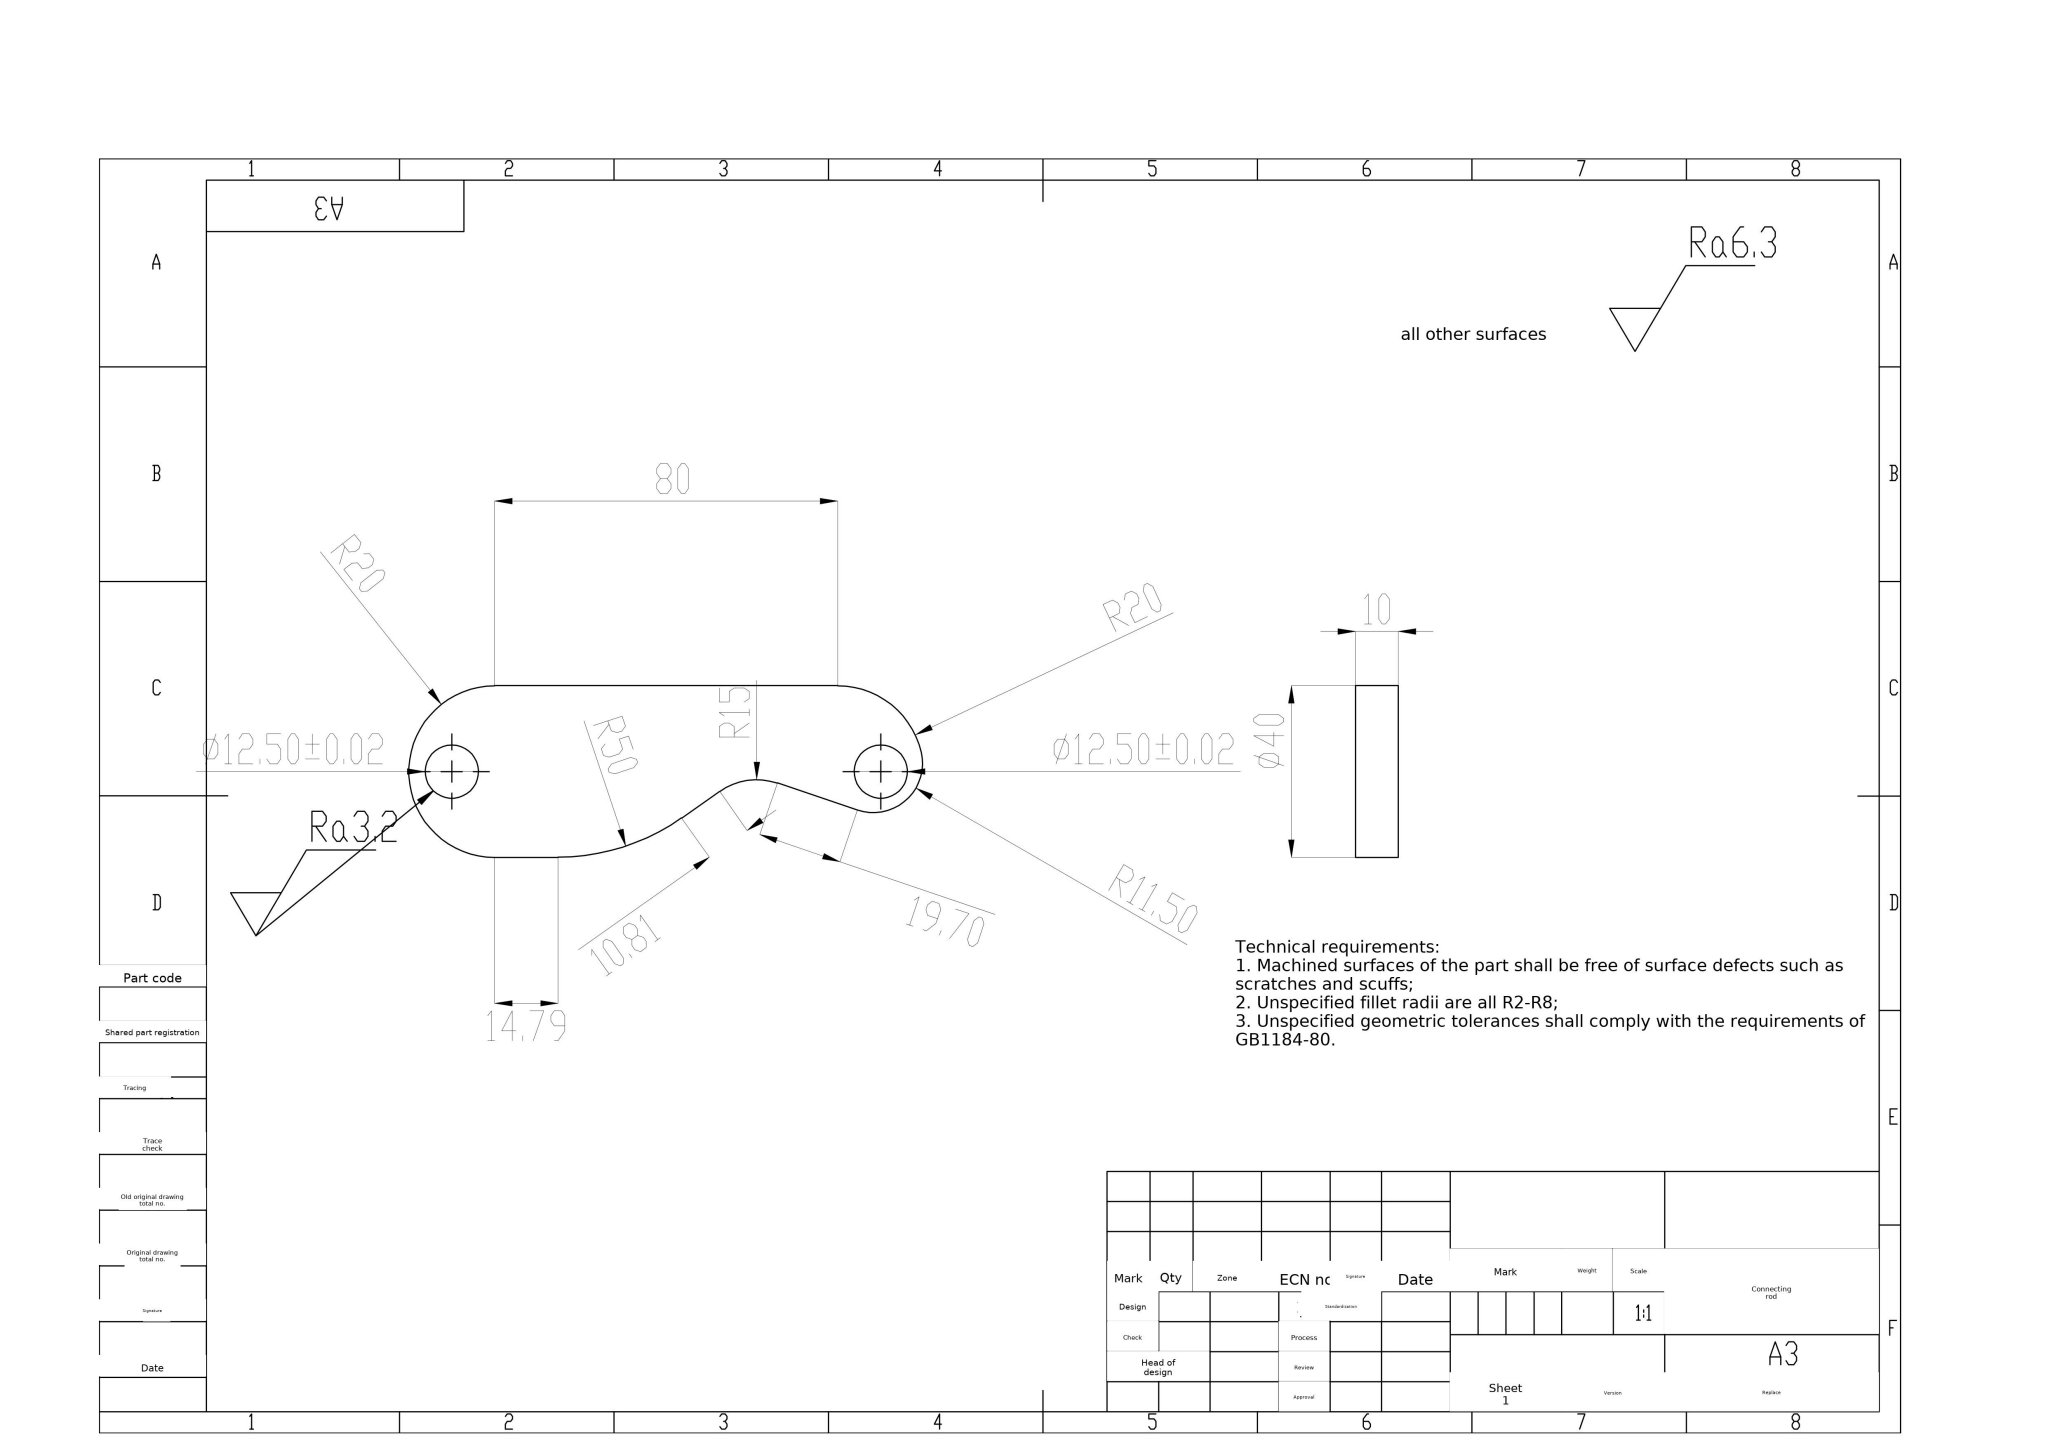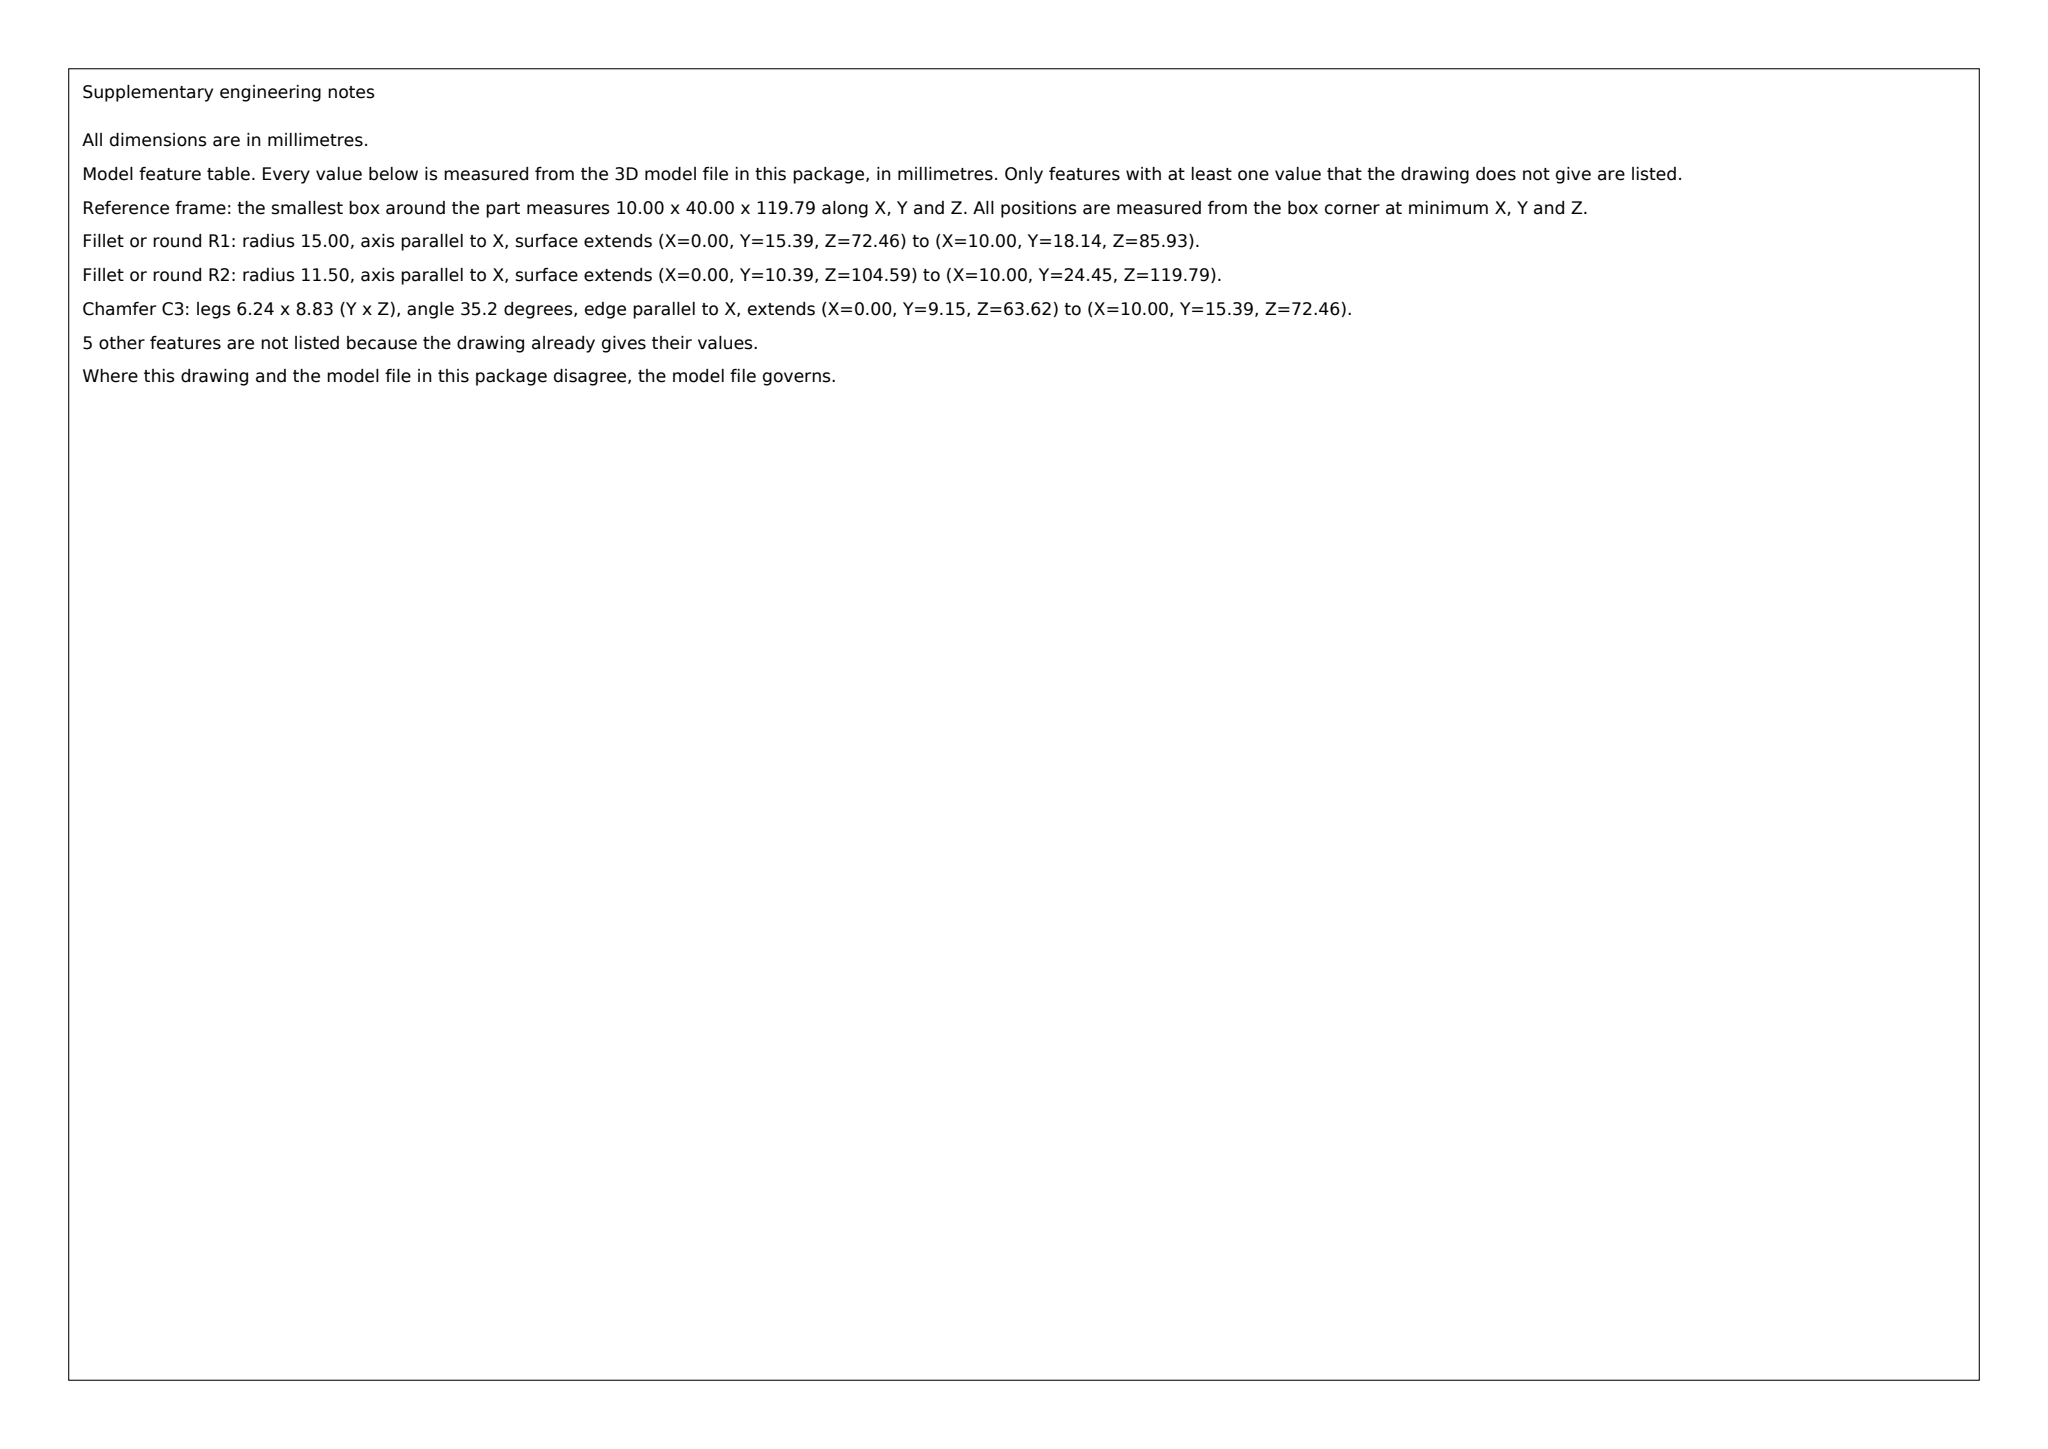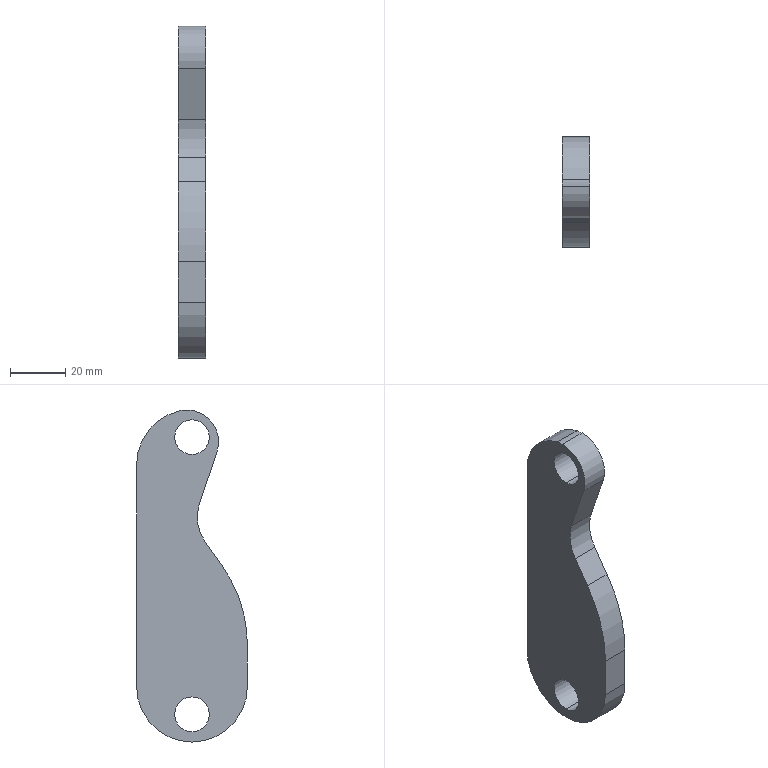Part | SolidWorks | mm | 1 solid | 16 faces | box 10 x 40 x 119.79 mm | volume 34125 mm3 | cylinder 10 | plane 6 | commonest cylinder face diameters 12.5 x4 23 x2 40 x2 30 x1 100 x1
build123d program:
from build123d import *

# Parameters (mm, degrees)
SKETCH1_R           = 1.25
BOSS_EXTRUDE1_DEPTH = 2
CUT_EXTRUDE1_DEPTH  = 13.806
FILLET1_R           = 10
FILLET2_R           = 2.3
SCALE1_SCALE        = 10
SCALE2_SCALE        = 10
SCALE3_SCALE        = 0.1
SCALE4_SCALE        = 0.5


with BuildPart() as part:
    # Sketch1 → Boss-Extrude1 (new body)
    with BuildSketch(Plane(origin=(0, 0, 0), x_dir=(0, 0, -1), z_dir=(1, 0, 0))):
        with BuildLine():
            Line((8, -4), (-8, -4))
            ThreePointArc((-8, -4), (-12, 0), (-8, 4))
            Line((-8, 4), (8, 4))
            ThreePointArc((8, 4), (12, 0), (8, -4))
        make_face()
        with Locations((10, 0)):
            Circle(SKETCH1_R, mode=Mode.SUBTRACT)
        with Locations(Location((-10, 0, 0), (0, 0, 180))):
            Circle(SKETCH1_R, mode=Mode.SUBTRACT)
    extrude(amount=BOSS_EXTRUDE1_DEPTH)

    # Sketch2 → Cut-Extrude1 (cut, through all)
    with BuildSketch(Plane.ZY):
        with BuildLine():
            Line((-1.868, -4), (2.491, -0.9222))
            ThreePointArc((2.491, -0.9222), (3.792, -0.4039), (5.186, -0.5324))
            Line((5.186, -0.5324), (13.896, -3.49))
            Line((13.896, -3.49), (11.205, -5.288))
            Line((11.205, -5.288), (0.9404, -6.462))
            Line((0.9404, -6.462), (-1.868, -4))
        make_face()
    extrude(amount=-CUT_EXTRUDE1_DEPTH, mode=Mode.SUBTRACT)

    # Fillet1
    fillet1_edges = [part.edges().sort_by_distance(p)[0] for p in [
        (1, -4, -1.868),
    ]]
    fillet(fillet1_edges, radius=FILLET1_R)

    # Fillet2
    fillet2_edges = [part.edges().sort_by_distance(p)[0] for p in [
        (1, -2.538, 11.092),
    ]]
    fillet(fillet2_edges, radius=FILLET2_R)


with BuildPart() as part_1:
    # Scale1: scaled about (1, 0.5999, -1.156)
    add(part.part.scale(SCALE1_SCALE).moved(Location((-9, -5.399, 10.403))))


with BuildPart() as part_2:
    # Scale2: scaled about (0, 0, 0)
    add(part_1.part.scale(SCALE2_SCALE))


with BuildPart() as part_3:
    # Scale3: scaled about (0, 0, 0)
    add(part_2.part.scale(SCALE3_SCALE))


with BuildPart() as part_4:
    # Scale4: scaled about (1, 0.5999, -1.156)
    add(part_3.part.scale(SCALE4_SCALE).moved(Location((0.5, 0.2999, -0.5779))))


solid = part_4.part
STEP:
#1=CARTESIAN_POINT('',(6.,-0.5085,64.41));
#2=VERTEX_POINT('',#1);
#3=CARTESIAN_POINT('',(6.,-11.398,49.212));
#4=VERTEX_POINT('',#3);
#5=CARTESIAN_POINT('',(6.,-0.5085,52.91));
#6=DIRECTION('',(1.,0.,-0.));
#7=DIRECTION('',(0.,-0.,-1.));
#8=AXIS2_PLACEMENT_3D('',#5,#6,#7);
#9=CIRCLE('',#8,11.5);
#10=EDGE_CURVE('',#2,#4,#9,.T.);
#11=ORIENTED_EDGE('',*,*,#10,.F.);
#12=CARTESIAN_POINT('',(-4.,-0.5085,64.41));
#13=VERTEX_POINT('',#12);
#14=CARTESIAN_POINT('',(6.,-0.5085,64.41));
#15=DIRECTION('',(-1.,-0.,0.));
#16=VECTOR('',#15,1000.);
#17=LINE('',#14,#16);
#18=EDGE_CURVE('',#2,#13,#17,.T.);
#19=ORIENTED_EDGE('',*,*,#18,.T.);
#20=CARTESIAN_POINT('',(-4.,-11.398,49.212));
#21=VERTEX_POINT('',#20);
#22=CARTESIAN_POINT('',(-4.,-0.5085,52.91));
#23=DIRECTION('',(-1.,-0.,0.));
#24=DIRECTION('',(0.,-0.,-1.));
#25=AXIS2_PLACEMENT_3D('',#22,#23,#24);
#26=CIRCLE('',#25,11.5);
#27=EDGE_CURVE('',#21,#13,#26,.T.);
#28=ORIENTED_EDGE('',*,*,#27,.F.);
#29=CARTESIAN_POINT('',(6.,-11.398,49.212));
#30=DIRECTION('',(-1.,-0.,0.));
#31=VECTOR('',#30,1000.);
#32=LINE('',#29,#31);
#33=EDGE_CURVE('',#4,#21,#32,.T.);
#34=ORIENTED_EDGE('',*,*,#33,.F.);
#35=EDGE_LOOP('',(#11,#19,#28,#34));
#36=FACE_OUTER_BOUND('',#35,.T.);
#37=CARTESIAN_POINT('',(6.,-0.5085,52.91));
#38=DIRECTION('',(-1.,-0.,0.));
#39=DIRECTION('',(0.,0.,1.));
#40=AXIS2_PLACEMENT_3D('',#37,#38,#39);
#41=CYLINDRICAL_SURFACE('',#40,11.5);
#42=ADVANCED_FACE('',(#36),#41,.T.);
#43=CARTESIAN_POINT('',(6.,-2.399,60.873));
#44=VERTEX_POINT('',#43);
#45=CARTESIAN_POINT('',(6.,-2.399,48.373));
#46=VERTEX_POINT('',#45);
#47=CARTESIAN_POINT('',(6.,-2.399,54.623));
#48=DIRECTION('',(1.,0.,-0.));
#49=DIRECTION('',(0.,0.,1.));
#50=AXIS2_PLACEMENT_3D('',#47,#48,#49);
#51=CIRCLE('',#50,6.25);
#52=EDGE_CURVE('',#44,#46,#51,.T.);
#53=ORIENTED_EDGE('',*,*,#52,.T.);
#54=CARTESIAN_POINT('',(-4.,-2.399,48.373));
#55=VERTEX_POINT('',#54);
#56=CARTESIAN_POINT('',(6.,-2.399,48.373));
#57=DIRECTION('',(-1.,-0.,0.));
#58=VECTOR('',#57,1000.);
#59=LINE('',#56,#58);
#60=EDGE_CURVE('',#46,#55,#59,.T.);
#61=ORIENTED_EDGE('',*,*,#60,.T.);
#62=CARTESIAN_POINT('',(-4.,-2.399,60.873));
#63=VERTEX_POINT('',#62);
#64=CARTESIAN_POINT('',(-4.,-2.399,54.623));
#65=DIRECTION('',(1.,0.,-0.));
#66=DIRECTION('',(0.,0.,1.));
#67=AXIS2_PLACEMENT_3D('',#64,#65,#66);
#68=CIRCLE('',#67,6.25);
#69=EDGE_CURVE('',#63,#55,#68,.T.);
#70=ORIENTED_EDGE('',*,*,#69,.F.);
#71=CARTESIAN_POINT('',(6.,-2.399,60.873));
#72=DIRECTION('',(-1.,-0.,0.));
#73=VECTOR('',#72,1000.);
#74=LINE('',#71,#73);
#75=EDGE_CURVE('',#44,#63,#74,.T.);
#76=ORIENTED_EDGE('',*,*,#75,.F.);
#77=EDGE_LOOP('',(#53,#61,#70,#76));
#78=FACE_OUTER_BOUND('',#77,.T.);
#79=CARTESIAN_POINT('',(6.,-2.399,54.623));
#80=DIRECTION('',(-1.,-0.,0.));
#81=DIRECTION('',(0.,0.,1.));
#82=AXIS2_PLACEMENT_3D('',#79,#80,#81);
#83=CYLINDRICAL_SURFACE('',#82,6.25);
#84=ADVANCED_FACE('',(#78),#83,.F.);
#85=CARTESIAN_POINT('',(6.,-2.399,-39.127));
#86=VERTEX_POINT('',#85);
#87=CARTESIAN_POINT('',(6.,-2.399,-51.627));
#88=VERTEX_POINT('',#87);
#89=CARTESIAN_POINT('',(6.,-2.399,-45.377));
#90=DIRECTION('',(1.,0.,-0.));
#91=DIRECTION('',(0.,-0.,-1.));
#92=AXIS2_PLACEMENT_3D('',#89,#90,#91);
#93=CIRCLE('',#92,6.25);
#94=EDGE_CURVE('',#86,#88,#93,.T.);
#95=ORIENTED_EDGE('',*,*,#94,.T.);
#96=CARTESIAN_POINT('',(-4.,-2.399,-51.627));
#97=VERTEX_POINT('',#96);
#98=CARTESIAN_POINT('',(6.,-2.399,-51.627));
#99=DIRECTION('',(-1.,-0.,0.));
#100=VECTOR('',#99,1000.);
#101=LINE('',#98,#100);
#102=EDGE_CURVE('',#88,#97,#101,.T.);
#103=ORIENTED_EDGE('',*,*,#102,.T.);
#104=CARTESIAN_POINT('',(-4.,-2.399,-39.127));
#105=VERTEX_POINT('',#104);
#106=CARTESIAN_POINT('',(-4.,-2.399,-45.377));
#107=DIRECTION('',(1.,0.,-0.));
#108=DIRECTION('',(0.,-0.,-1.));
#109=AXIS2_PLACEMENT_3D('',#106,#107,#108);
#110=CIRCLE('',#109,6.25);
#111=EDGE_CURVE('',#105,#97,#110,.T.);
#112=ORIENTED_EDGE('',*,*,#111,.F.);
#113=CARTESIAN_POINT('',(6.,-2.399,-39.127));
#114=DIRECTION('',(-1.,-0.,0.));
#115=VECTOR('',#114,1000.);
#116=LINE('',#113,#115);
#117=EDGE_CURVE('',#86,#105,#116,.T.);
#118=ORIENTED_EDGE('',*,*,#117,.F.);
#119=EDGE_LOOP('',(#95,#103,#112,#118));
#120=FACE_OUTER_BOUND('',#119,.T.);
#121=CARTESIAN_POINT('',(6.,-2.399,-45.377));
#122=DIRECTION('',(-1.,-0.,0.));
#123=DIRECTION('',(0.,0.,1.));
#124=AXIS2_PLACEMENT_3D('',#121,#122,#123);
#125=CYLINDRICAL_SURFACE('',#124,6.25);
#126=ADVANCED_FACE('',(#120),#125,.F.);
#127=CARTESIAN_POINT('',(6.,17.601,44.623));
#128=VERTEX_POINT('',#127);
#129=CARTESIAN_POINT('',(6.,2.05,64.122));
#130=VERTEX_POINT('',#129);
#131=CARTESIAN_POINT('',(6.,-2.399,44.623));
#132=DIRECTION('',(1.,0.,-0.));
#133=DIRECTION('',(-0.,0.,1.));
#134=AXIS2_PLACEMENT_3D('',#131,#132,#133);
#135=CIRCLE('',#134,20.);
#136=EDGE_CURVE('',#128,#130,#135,.T.);
#137=ORIENTED_EDGE('',*,*,#136,.T.);
#138=CARTESIAN_POINT('',(6.,-0.5085,52.91));
#139=DIRECTION('',(1.,0.,-0.));
#140=DIRECTION('',(0.,-0.,-1.));
#141=AXIS2_PLACEMENT_3D('',#138,#139,#140);
#142=CIRCLE('',#141,11.5);
#143=EDGE_CURVE('',#130,#2,#142,.T.);
#144=ORIENTED_EDGE('',*,*,#143,.T.);
#145=ORIENTED_EDGE('',*,*,#10,.T.);
#146=CARTESIAN_POINT('',(6.,-5.061,30.556));
#147=VERTEX_POINT('',#146);
#148=CARTESIAN_POINT('',(6.,-5.061,30.556));
#149=DIRECTION('',(0.,0.3216,-0.9469));
#150=VECTOR('',#149,1000.);
#151=LINE('',#148,#150);
#152=EDGE_CURVE('',#4,#147,#151,.T.);
#153=ORIENTED_EDGE('',*,*,#152,.T.);
#154=CARTESIAN_POINT('',(6.,-7.011,17.081));
#155=VERTEX_POINT('',#154);
#156=CARTESIAN_POINT('',(6.,-19.264,25.732));
#157=DIRECTION('',(-1.,-0.,0.));
#158=DIRECTION('',(0.,0.,1.));
#159=AXIS2_PLACEMENT_3D('',#156,#157,#158);
#160=CIRCLE('',#159,15.);
#161=EDGE_CURVE('',#147,#155,#160,.T.);
#162=ORIENTED_EDGE('',*,*,#161,.T.);
#163=CARTESIAN_POINT('',(6.,-13.246,8.248));
#164=VERTEX_POINT('',#163);
#165=CARTESIAN_POINT('',(6.,-22.399,-4.717));
#166=DIRECTION('',(0.,-0.5767,-0.8169));
#167=VECTOR('',#166,1000.);
#168=LINE('',#165,#167);
#169=EDGE_CURVE('',#155,#164,#168,.T.);
#170=ORIENTED_EDGE('',*,*,#169,.T.);
#171=CARTESIAN_POINT('',(6.,-22.399,-20.588));
#172=VERTEX_POINT('',#171);
#173=CARTESIAN_POINT('',(6.,27.601,-20.588));
#174=DIRECTION('',(1.,0.,-0.));
#175=DIRECTION('',(0.,-0.,-1.));
#176=AXIS2_PLACEMENT_3D('',#173,#174,#175);
#177=CIRCLE('',#176,50.);
#178=EDGE_CURVE('',#164,#172,#177,.T.);
#179=ORIENTED_EDGE('',*,*,#178,.T.);
#180=CARTESIAN_POINT('',(6.,-22.399,-35.377));
#181=VERTEX_POINT('',#180);
#182=CARTESIAN_POINT('',(6.,-22.399,-35.377));
#183=DIRECTION('',(0.,-0.,-1.));
#184=VECTOR('',#183,1000.);
#185=LINE('',#182,#184);
#186=EDGE_CURVE('',#172,#181,#185,.T.);
#187=ORIENTED_EDGE('',*,*,#186,.T.);
#188=CARTESIAN_POINT('',(6.,17.601,-35.377));
#189=VERTEX_POINT('',#188);
#190=CARTESIAN_POINT('',(6.,-2.399,-35.377));
#191=DIRECTION('',(1.,0.,-0.));
#192=DIRECTION('',(0.,-0.,-1.));
#193=AXIS2_PLACEMENT_3D('',#190,#191,#192);
#194=CIRCLE('',#193,20.);
#195=EDGE_CURVE('',#181,#189,#194,.T.);
#196=ORIENTED_EDGE('',*,*,#195,.T.);
#197=CARTESIAN_POINT('',(6.,17.601,-35.377));
#198=DIRECTION('',(-0.,0.,1.));
#199=VECTOR('',#198,1000.);
#200=LINE('',#197,#199);
#201=EDGE_CURVE('',#189,#128,#200,.T.);
#202=ORIENTED_EDGE('',*,*,#201,.T.);
#203=EDGE_LOOP('',(#137,#144,#145,#153,#162,#170,#179,#187,#196,#202));
#204=FACE_OUTER_BOUND('',#203,.T.);
#205=ORIENTED_EDGE('',*,*,#94,.F.);
#206=CARTESIAN_POINT('',(6.,-2.399,-45.377));
#207=DIRECTION('',(1.,0.,-0.));
#208=DIRECTION('',(0.,-0.,-1.));
#209=AXIS2_PLACEMENT_3D('',#206,#207,#208);
#210=CIRCLE('',#209,6.25);
#211=EDGE_CURVE('',#88,#86,#210,.T.);
#212=ORIENTED_EDGE('',*,*,#211,.F.);
#213=EDGE_LOOP('',(#205,#212));
#214=FACE_BOUND('',#213,.T.);
#215=ORIENTED_EDGE('',*,*,#52,.F.);
#216=CARTESIAN_POINT('',(6.,-2.399,54.623));
#217=DIRECTION('',(1.,0.,-0.));
#218=DIRECTION('',(0.,0.,1.));
#219=AXIS2_PLACEMENT_3D('',#216,#217,#218);
#220=CIRCLE('',#219,6.25);
#221=EDGE_CURVE('',#46,#44,#220,.T.);
#222=ORIENTED_EDGE('',*,*,#221,.F.);
#223=EDGE_LOOP('',(#215,#222));
#224=FACE_BOUND('',#223,.T.);
#225=CARTESIAN_POINT('',(6.,-2.399,-35.377));
#226=DIRECTION('',(1.,0.,0.));
#227=DIRECTION('',(0.,-0.,-1.));
#228=AXIS2_PLACEMENT_3D('',#225,#226,#227);
#229=PLANE('',#228);
#230=ADVANCED_FACE('',(#204,#214,#224),#229,.T.);
#231=CARTESIAN_POINT('',(-4.,-5.061,30.556));
#232=VERTEX_POINT('',#231);
#233=CARTESIAN_POINT('',(-4.,-5.061,30.556));
#234=DIRECTION('',(0.,0.3216,-0.9469));
#235=VECTOR('',#234,1000.);
#236=LINE('',#233,#235);
#237=EDGE_CURVE('',#21,#232,#236,.T.);
#238=ORIENTED_EDGE('',*,*,#237,.F.);
#239=ORIENTED_EDGE('',*,*,#27,.T.);
#240=CARTESIAN_POINT('',(-4.,2.05,64.122));
#241=VERTEX_POINT('',#240);
#242=CARTESIAN_POINT('',(-4.,-0.5085,52.91));
#243=DIRECTION('',(-1.,-0.,0.));
#244=DIRECTION('',(0.,0.,-1.));
#245=AXIS2_PLACEMENT_3D('',#242,#243,#244);
#246=CIRCLE('',#245,11.5);
#247=EDGE_CURVE('',#13,#241,#246,.T.);
#248=ORIENTED_EDGE('',*,*,#247,.T.);
#249=CARTESIAN_POINT('',(-4.,17.601,44.623));
#250=VERTEX_POINT('',#249);
#251=CARTESIAN_POINT('',(-4.,-2.399,44.623));
#252=DIRECTION('',(1.,0.,-0.));
#253=DIRECTION('',(-0.,0.,1.));
#254=AXIS2_PLACEMENT_3D('',#251,#252,#253);
#255=CIRCLE('',#254,20.);
#256=EDGE_CURVE('',#250,#241,#255,.T.);
#257=ORIENTED_EDGE('',*,*,#256,.F.);
#258=CARTESIAN_POINT('',(-4.,17.601,-35.377));
#259=VERTEX_POINT('',#258);
#260=CARTESIAN_POINT('',(-4.,17.601,-35.377));
#261=DIRECTION('',(-0.,0.,1.));
#262=VECTOR('',#261,1000.);
#263=LINE('',#260,#262);
#264=EDGE_CURVE('',#259,#250,#263,.T.);
#265=ORIENTED_EDGE('',*,*,#264,.F.);
#266=CARTESIAN_POINT('',(-4.,-22.399,-35.377));
#267=VERTEX_POINT('',#266);
#268=CARTESIAN_POINT('',(-4.,-2.399,-35.377));
#269=DIRECTION('',(1.,0.,-0.));
#270=DIRECTION('',(0.,-0.,-1.));
#271=AXIS2_PLACEMENT_3D('',#268,#269,#270);
#272=CIRCLE('',#271,20.);
#273=EDGE_CURVE('',#267,#259,#272,.T.);
#274=ORIENTED_EDGE('',*,*,#273,.F.);
#275=CARTESIAN_POINT('',(-4.,-22.399,-20.588));
#276=VERTEX_POINT('',#275);
#277=CARTESIAN_POINT('',(-4.,-22.399,-35.377));
#278=DIRECTION('',(0.,-0.,-1.));
#279=VECTOR('',#278,1000.);
#280=LINE('',#277,#279);
#281=EDGE_CURVE('',#276,#267,#280,.T.);
#282=ORIENTED_EDGE('',*,*,#281,.F.);
#283=CARTESIAN_POINT('',(-4.,-13.246,8.248));
#284=VERTEX_POINT('',#283);
#285=CARTESIAN_POINT('',(-4.,27.601,-20.588));
#286=DIRECTION('',(-1.,-0.,0.));
#287=DIRECTION('',(0.,-0.,-1.));
#288=AXIS2_PLACEMENT_3D('',#285,#286,#287);
#289=CIRCLE('',#288,50.);
#290=EDGE_CURVE('',#276,#284,#289,.T.);
#291=ORIENTED_EDGE('',*,*,#290,.T.);
#292=CARTESIAN_POINT('',(-4.,-7.011,17.081));
#293=VERTEX_POINT('',#292);
#294=CARTESIAN_POINT('',(-4.,-22.399,-4.717));
#295=DIRECTION('',(0.,-0.5767,-0.8169));
#296=VECTOR('',#295,1000.);
#297=LINE('',#294,#296);
#298=EDGE_CURVE('',#293,#284,#297,.T.);
#299=ORIENTED_EDGE('',*,*,#298,.F.);
#300=CARTESIAN_POINT('',(-4.,-19.264,25.732));
#301=DIRECTION('',(-1.,-0.,0.));
#302=DIRECTION('',(0.,0.,1.));
#303=AXIS2_PLACEMENT_3D('',#300,#301,#302);
#304=CIRCLE('',#303,15.);
#305=EDGE_CURVE('',#232,#293,#304,.T.);
#306=ORIENTED_EDGE('',*,*,#305,.F.);
#307=EDGE_LOOP('',(#238,#239,#248,#257,#265,#274,#282,#291,#299,#306));
#308=FACE_OUTER_BOUND('',#307,.T.);
#309=ORIENTED_EDGE('',*,*,#111,.T.);
#310=CARTESIAN_POINT('',(-4.,-2.399,-45.377));
#311=DIRECTION('',(1.,0.,-0.));
#312=DIRECTION('',(0.,-0.,-1.));
#313=AXIS2_PLACEMENT_3D('',#310,#311,#312);
#314=CIRCLE('',#313,6.25);
#315=EDGE_CURVE('',#97,#105,#314,.T.);
#316=ORIENTED_EDGE('',*,*,#315,.T.);
#317=EDGE_LOOP('',(#309,#316));
#318=FACE_BOUND('',#317,.T.);
#319=ORIENTED_EDGE('',*,*,#69,.T.);
#320=CARTESIAN_POINT('',(-4.,-2.399,54.623));
#321=DIRECTION('',(1.,0.,-0.));
#322=DIRECTION('',(0.,0.,1.));
#323=AXIS2_PLACEMENT_3D('',#320,#321,#322);
#324=CIRCLE('',#323,6.25);
#325=EDGE_CURVE('',#55,#63,#324,.T.);
#326=ORIENTED_EDGE('',*,*,#325,.T.);
#327=EDGE_LOOP('',(#319,#326));
#328=FACE_BOUND('',#327,.T.);
#329=CARTESIAN_POINT('',(-4.,-2.399,-35.377));
#330=DIRECTION('',(1.,0.,0.));
#331=DIRECTION('',(0.,-0.,-1.));
#332=AXIS2_PLACEMENT_3D('',#329,#330,#331);
#333=PLANE('',#332);
#334=ADVANCED_FACE('',(#308,#318,#328),#333,.F.);
#335=ORIENTED_EDGE('',*,*,#273,.T.);
#336=CARTESIAN_POINT('',(6.,17.601,-35.377));
#337=DIRECTION('',(-1.,-0.,0.));
#338=VECTOR('',#337,1000.);
#339=LINE('',#336,#338);
#340=EDGE_CURVE('',#189,#259,#339,.T.);
#341=ORIENTED_EDGE('',*,*,#340,.F.);
#342=ORIENTED_EDGE('',*,*,#195,.F.);
#343=CARTESIAN_POINT('',(6.,-22.399,-35.377));
#344=DIRECTION('',(-1.,-0.,0.));
#345=VECTOR('',#344,1000.);
#346=LINE('',#343,#345);
#347=EDGE_CURVE('',#181,#267,#346,.T.);
#348=ORIENTED_EDGE('',*,*,#347,.T.);
#349=EDGE_LOOP('',(#335,#341,#342,#348));
#350=FACE_OUTER_BOUND('',#349,.T.);
#351=CARTESIAN_POINT('',(6.,-2.399,-35.377));
#352=DIRECTION('',(-1.,-0.,0.));
#353=DIRECTION('',(-0.,0.,1.));
#354=AXIS2_PLACEMENT_3D('',#351,#352,#353);
#355=CYLINDRICAL_SURFACE('',#354,20.);
#356=ADVANCED_FACE('',(#350),#355,.T.);
#357=ORIENTED_EDGE('',*,*,#264,.T.);
#358=CARTESIAN_POINT('',(6.,17.601,44.623));
#359=DIRECTION('',(-1.,-0.,0.));
#360=VECTOR('',#359,1000.);
#361=LINE('',#358,#360);
#362=EDGE_CURVE('',#128,#250,#361,.T.);
#363=ORIENTED_EDGE('',*,*,#362,.F.);
#364=ORIENTED_EDGE('',*,*,#201,.F.);
#365=ORIENTED_EDGE('',*,*,#340,.T.);
#366=EDGE_LOOP('',(#357,#363,#364,#365));
#367=FACE_OUTER_BOUND('',#366,.T.);
#368=CARTESIAN_POINT('',(6.,17.601,-35.377));
#369=DIRECTION('',(0.,-1.,0.));
#370=DIRECTION('',(0.,-0.,-1.));
#371=AXIS2_PLACEMENT_3D('',#368,#369,#370);
#372=PLANE('',#371);
#373=ADVANCED_FACE('',(#367),#372,.F.);
#374=ORIENTED_EDGE('',*,*,#256,.T.);
#375=CARTESIAN_POINT('',(6.,2.05,64.122));
#376=DIRECTION('',(1.,0.,-0.));
#377=VECTOR('',#376,1000.);
#378=LINE('',#375,#377);
#379=EDGE_CURVE('',#241,#130,#378,.T.);
#380=ORIENTED_EDGE('',*,*,#379,.T.);
#381=ORIENTED_EDGE('',*,*,#136,.F.);
#382=ORIENTED_EDGE('',*,*,#362,.T.);
#383=EDGE_LOOP('',(#374,#380,#381,#382));
#384=FACE_OUTER_BOUND('',#383,.T.);
#385=CARTESIAN_POINT('',(6.,-2.399,44.623));
#386=DIRECTION('',(-1.,-0.,0.));
#387=DIRECTION('',(-0.,0.,1.));
#388=AXIS2_PLACEMENT_3D('',#385,#386,#387);
#389=CYLINDRICAL_SURFACE('',#388,20.);
#390=ADVANCED_FACE('',(#384),#389,.T.);
#391=ORIENTED_EDGE('',*,*,#186,.F.);
#392=CARTESIAN_POINT('',(6.,-22.399,-20.588));
#393=DIRECTION('',(-1.,-0.,0.));
#394=VECTOR('',#393,1000.);
#395=LINE('',#392,#394);
#396=EDGE_CURVE('',#172,#276,#395,.T.);
#397=ORIENTED_EDGE('',*,*,#396,.T.);
#398=ORIENTED_EDGE('',*,*,#281,.T.);
#399=ORIENTED_EDGE('',*,*,#347,.F.);
#400=EDGE_LOOP('',(#391,#397,#398,#399));
#401=FACE_OUTER_BOUND('',#400,.T.);
#402=CARTESIAN_POINT('',(6.,-22.399,-35.377));
#403=DIRECTION('',(-0.,1.,-0.));
#404=DIRECTION('',(-0.,0.,1.));
#405=AXIS2_PLACEMENT_3D('',#402,#403,#404);
#406=PLANE('',#405);
#407=ADVANCED_FACE('',(#401),#406,.F.);
#408=ORIENTED_EDGE('',*,*,#102,.F.);
#409=ORIENTED_EDGE('',*,*,#211,.T.);
#410=ORIENTED_EDGE('',*,*,#117,.T.);
#411=ORIENTED_EDGE('',*,*,#315,.F.);
#412=EDGE_LOOP('',(#408,#409,#410,#411));
#413=FACE_OUTER_BOUND('',#412,.T.);
#414=CARTESIAN_POINT('',(6.,-2.399,-45.377));
#415=DIRECTION('',(-1.,-0.,0.));
#416=DIRECTION('',(0.,0.,1.));
#417=AXIS2_PLACEMENT_3D('',#414,#415,#416);
#418=CYLINDRICAL_SURFACE('',#417,6.25);
#419=ADVANCED_FACE('',(#413),#418,.F.);
#420=ORIENTED_EDGE('',*,*,#60,.F.);
#421=ORIENTED_EDGE('',*,*,#221,.T.);
#422=ORIENTED_EDGE('',*,*,#75,.T.);
#423=ORIENTED_EDGE('',*,*,#325,.F.);
#424=EDGE_LOOP('',(#420,#421,#422,#423));
#425=FACE_OUTER_BOUND('',#424,.T.);
#426=CARTESIAN_POINT('',(6.,-2.399,54.623));
#427=DIRECTION('',(-1.,-0.,0.));
#428=DIRECTION('',(0.,0.,1.));
#429=AXIS2_PLACEMENT_3D('',#426,#427,#428);
#430=CYLINDRICAL_SURFACE('',#429,6.25);
#431=ADVANCED_FACE('',(#425),#430,.F.);
#432=ORIENTED_EDGE('',*,*,#152,.F.);
#433=ORIENTED_EDGE('',*,*,#33,.T.);
#434=ORIENTED_EDGE('',*,*,#237,.T.);
#435=CARTESIAN_POINT('',(6.,-5.061,30.556));
#436=DIRECTION('',(-1.,-0.,0.));
#437=VECTOR('',#436,1000.);
#438=LINE('',#435,#437);
#439=EDGE_CURVE('',#147,#232,#438,.T.);
#440=ORIENTED_EDGE('',*,*,#439,.F.);
#441=EDGE_LOOP('',(#432,#433,#434,#440));
#442=FACE_OUTER_BOUND('',#441,.T.);
#443=CARTESIAN_POINT('',(6.,-5.061,30.556));
#444=DIRECTION('',(-0.,0.9469,0.3216));
#445=DIRECTION('',(-0.,-0.3216,0.9469));
#446=AXIS2_PLACEMENT_3D('',#443,#444,#445);
#447=PLANE('',#446);
#448=ADVANCED_FACE('',(#442),#447,.F.);
#449=ORIENTED_EDGE('',*,*,#298,.T.);
#450=CARTESIAN_POINT('',(6.,-13.246,8.248));
#451=DIRECTION('',(1.,0.,-0.));
#452=VECTOR('',#451,1000.);
#453=LINE('',#450,#452);
#454=EDGE_CURVE('',#284,#164,#453,.T.);
#455=ORIENTED_EDGE('',*,*,#454,.T.);
#456=ORIENTED_EDGE('',*,*,#169,.F.);
#457=CARTESIAN_POINT('',(6.,-7.011,17.081));
#458=DIRECTION('',(-1.,-0.,0.));
#459=VECTOR('',#458,1000.);
#460=LINE('',#457,#459);
#461=EDGE_CURVE('',#155,#293,#460,.T.);
#462=ORIENTED_EDGE('',*,*,#461,.T.);
#463=EDGE_LOOP('',(#449,#455,#456,#462));
#464=FACE_OUTER_BOUND('',#463,.T.);
#465=CARTESIAN_POINT('',(6.,-22.399,-4.717));
#466=DIRECTION('',(-0.,0.8169,-0.5767));
#467=DIRECTION('',(-0.,0.5767,0.8169));
#468=AXIS2_PLACEMENT_3D('',#465,#466,#467);
#469=PLANE('',#468);
#470=ADVANCED_FACE('',(#464),#469,.F.);
#471=ORIENTED_EDGE('',*,*,#305,.T.);
#472=ORIENTED_EDGE('',*,*,#461,.F.);
#473=ORIENTED_EDGE('',*,*,#161,.F.);
#474=ORIENTED_EDGE('',*,*,#439,.T.);
#475=EDGE_LOOP('',(#471,#472,#473,#474));
#476=FACE_OUTER_BOUND('',#475,.T.);
#477=CARTESIAN_POINT('',(6.,-19.264,25.732));
#478=DIRECTION('',(-1.,-0.,0.));
#479=DIRECTION('',(0.,0.,1.));
#480=AXIS2_PLACEMENT_3D('',#477,#478,#479);
#481=CYLINDRICAL_SURFACE('',#480,15.);
#482=ADVANCED_FACE('',(#476),#481,.F.);
#483=ORIENTED_EDGE('',*,*,#178,.F.);
#484=ORIENTED_EDGE('',*,*,#454,.F.);
#485=ORIENTED_EDGE('',*,*,#290,.F.);
#486=ORIENTED_EDGE('',*,*,#396,.F.);
#487=EDGE_LOOP('',(#483,#484,#485,#486));
#488=FACE_OUTER_BOUND('',#487,.T.);
#489=CARTESIAN_POINT('',(6.,27.601,-20.588));
#490=DIRECTION('',(-1.,-0.,0.));
#491=DIRECTION('',(-0.,0.,1.));
#492=AXIS2_PLACEMENT_3D('',#489,#490,#491);
#493=CYLINDRICAL_SURFACE('',#492,50.);
#494=ADVANCED_FACE('',(#488),#493,.T.);
#495=ORIENTED_EDGE('',*,*,#18,.F.);
#496=ORIENTED_EDGE('',*,*,#143,.F.);
#497=ORIENTED_EDGE('',*,*,#379,.F.);
#498=ORIENTED_EDGE('',*,*,#247,.F.);
#499=EDGE_LOOP('',(#495,#496,#497,#498));
#500=FACE_OUTER_BOUND('',#499,.T.);
#501=CARTESIAN_POINT('',(6.,-0.5085,52.91));
#502=DIRECTION('',(-1.,-0.,0.));
#503=DIRECTION('',(0.,0.,1.));
#504=AXIS2_PLACEMENT_3D('',#501,#502,#503);
#505=CYLINDRICAL_SURFACE('',#504,11.5);
#506=ADVANCED_FACE('',(#500),#505,.T.);
#507=CLOSED_SHELL('',(#42,#84,#126,#230,#334,#356,#373,#390,#407,#419,#431,#448,#470,#482,#494,#506));
#508=MANIFOLD_SOLID_BREP('',#507);
#509=CARTESIAN_POINT('',(0.,0.,0.));
#510=DIRECTION('',(0.,0.,1.));
#511=DIRECTION('',(1.,0.,0.));
#512=AXIS2_PLACEMENT_3D('',#509,#510,#511);
#513=(LENGTH_UNIT()NAMED_UNIT(*)SI_UNIT(.MILLI.,.METRE.));
#514=UNCERTAINTY_MEASURE_WITH_UNIT(LENGTH_MEASURE(0.00001),#513,'','');
#515=(NAMED_UNIT(*)PLANE_ANGLE_UNIT()SI_UNIT($,.RADIAN.));
#516=(NAMED_UNIT(*)SI_UNIT($,.STERADIAN.)SOLID_ANGLE_UNIT());
#517=(GEOMETRIC_REPRESENTATION_CONTEXT(3)GLOBAL_UNCERTAINTY_ASSIGNED_CONTEXT((#514))GLOBAL_UNIT_ASSIGNED_CONTEXT((#513,#515,#516))REPRESENTATION_CONTEXT('',''));
#518=ADVANCED_BREP_SHAPE_REPRESENTATION('',(#508,#512),#517);